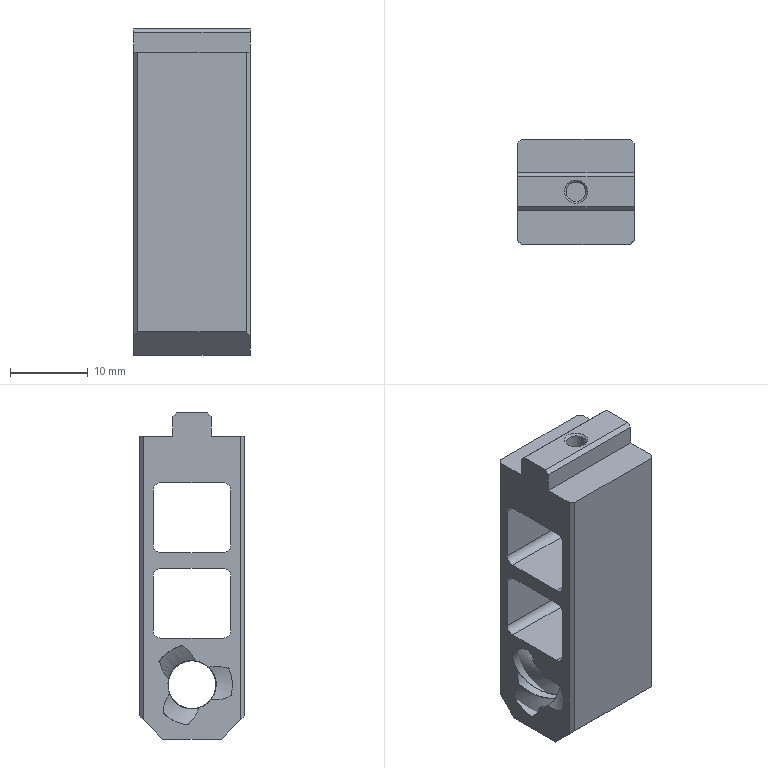Component | NX | DJZ_12_JAW_NUT_LH_2 | 1 solid | 52 faces | volume 4387 mm3 | plane 26 | spline 12 | cylinder 12 | cone 2 | commonest cylinder face diameters 2 x8 6.2 x3 2.5 x1